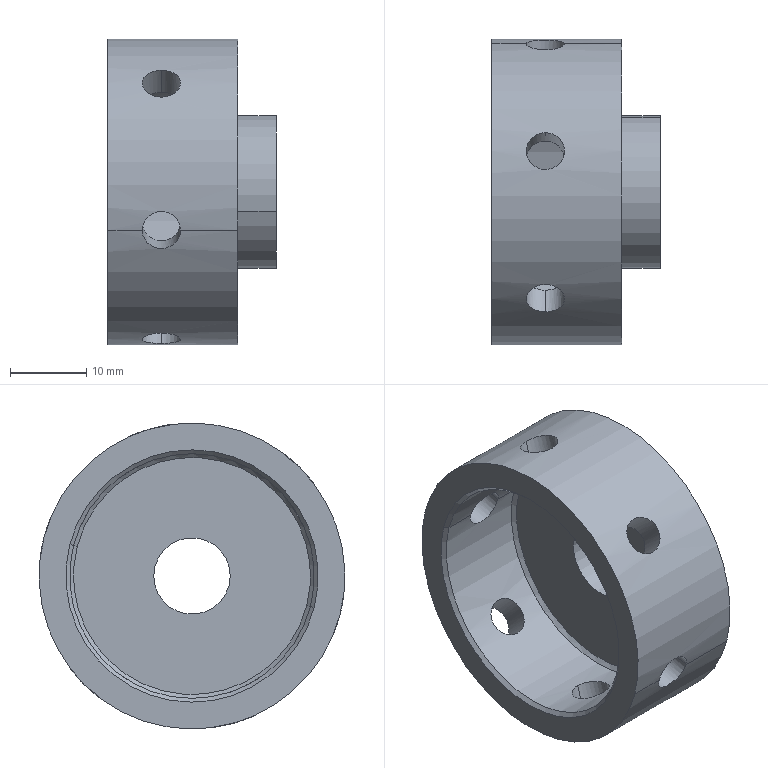Component | SolidWorks | 13LargeKnurledNut-1 | 1 solid | 30 faces | volume 11299 mm3 | cylinder 20 | cone 6 | plane 4 | commonest cylinder face diameters 5 x12 32 x2 20 x2 40 x2 10 x2